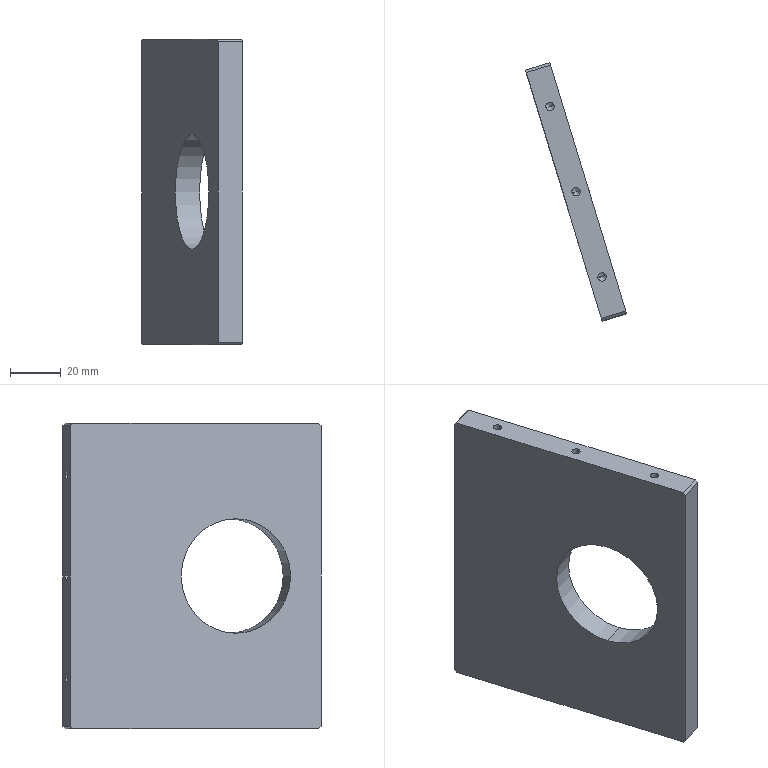Component | SolidWorks | V1ZHXTGrindingBasePlateReinforcementRibSB1-1 | 1 solid | 36 faces | box 39.62 x 101.43 x 120 mm | volume 107140 mm3 | cylinder 14 | cone 12 | plane 10 | commonest cylinder face diameters 3.3 x12 45 x2
build123d program:
from build123d import *

# Parameters (mm, degrees)
SKETCH1_W             = 120
SKETCH1_H             = 103
BOSS_EXTRUDE1_DEPTH   = 5
M4_TAPPED_HOLE1_D     = 3.3
M4_TAPPED_HOLE1_DEPTH = 10.1
M4_TAPPED_HOLE1_TIP   = 0.9914
M4_TAPPED_HOLE2_D     = 3.3
M4_TAPPED_HOLE2_DEPTH = 10.1
M4_TAPPED_HOLE2_TIP   = 0.9914
SKETCH7_R             = 22.5
CUT_EXTRUDE1_DEPTH    = 10
CHAMFER1_SIZE         = 1


with BuildPart() as part:
    # Sketch1 → Boss-Extrude1 (new, symmetric)
    with BuildSketch(Plane.XY):
        Rectangle(SKETCH1_W, SKETCH1_H)
    extrude(amount=BOSS_EXTRUDE1_DEPTH, both=True)

    # M4 Tapped Hole1
    with Locations(Plane.ZY.offset(60)):
        with Locations((0, 35), (0, 0), (0, -35)):
            Hole(M4_TAPPED_HOLE1_D / 2, depth=M4_TAPPED_HOLE1_DEPTH)
            with Locations((0, 0, -(M4_TAPPED_HOLE1_DEPTH + M4_TAPPED_HOLE1_TIP / 2))):  # 118° drill point
                Cone(0, M4_TAPPED_HOLE1_D / 2, M4_TAPPED_HOLE1_TIP, mode=Mode.SUBTRACT)

    # M4 Tapped Hole2
    with Locations(Plane(origin=(0, -51.5, 0), x_dir=(-1, 0, 0), z_dir=(0, -1, 0))):
        with Locations((40, 0), (0, 0), (-40, 0)):
            Hole(M4_TAPPED_HOLE2_D / 2, depth=M4_TAPPED_HOLE2_DEPTH)
            with Locations((0, 0, -(M4_TAPPED_HOLE2_DEPTH + M4_TAPPED_HOLE2_TIP / 2))):  # 118° drill point
                Cone(0, M4_TAPPED_HOLE2_D / 2, M4_TAPPED_HOLE2_TIP, mode=Mode.SUBTRACT)

    # Sketch7 → Cut-Extrude1 (cut)
    with BuildSketch(Plane.XY.offset(5)):
        with Locations((0, 16.5)):
            Circle(SKETCH7_R)
    extrude(amount=-CUT_EXTRUDE1_DEPTH, mode=Mode.SUBTRACT)

    # Chamfer1
    chamfer1_edges = [part.edges().sort_by_distance(p)[0] for p in [
        (60, -51.5, 0),
        (-60, -51.5, 0),
        (-60, 51.5, 0),
        (60, 51.5, 0),
    ]]
    chamfer(chamfer1_edges, length=CHAMFER1_SIZE)


solid = part.part

# Placed as in the assembly
solid = solid.moved(Location((244.147, -194.476, 375.239), (90, -73.032, -90)))
STEP:
#1=CARTESIAN_POINT('',(9.99,-8.22,15.659));
#2=VERTEX_POINT('',#1);
#3=CARTESIAN_POINT('',(9.99,-8.22,13.887));
#4=VERTEX_POINT('',#3);
#5=CARTESIAN_POINT('',(9.99,-8.22,14.773));
#6=DIRECTION('',(-0.9565,-0.2918,-0.));
#7=DIRECTION('',(0.,0.,-1.));
#8=AXIS2_PLACEMENT_3D('',#5,#6,#7);
#9=CIRCLE('',#8,0.8858);
#10=EDGE_CURVE('',#2,#4,#9,.T.);
#11=ORIENTED_EDGE('',*,*,#10,.F.);
#12=CARTESIAN_POINT('',(9.613,-8.335,15.659));
#13=VERTEX_POINT('',#12);
#14=CARTESIAN_POINT('',(9.99,-8.22,15.659));
#15=DIRECTION('',(-0.9565,-0.2918,-0.));
#16=VECTOR('',#15,39.37);
#17=LINE('',#14,#16);
#18=EDGE_CURVE('',#2,#13,#17,.T.);
#19=ORIENTED_EDGE('',*,*,#18,.T.);
#20=CARTESIAN_POINT('',(9.613,-8.335,13.887));
#21=VERTEX_POINT('',#20);
#22=CARTESIAN_POINT('',(9.613,-8.335,14.773));
#23=DIRECTION('',(-0.9565,-0.2918,-0.));
#24=DIRECTION('',(0.,0.,-1.));
#25=AXIS2_PLACEMENT_3D('',#22,#23,#24);
#26=CIRCLE('',#25,0.8858);
#27=EDGE_CURVE('',#13,#21,#26,.T.);
#28=ORIENTED_EDGE('',*,*,#27,.T.);
#29=CARTESIAN_POINT('',(9.99,-8.22,13.887));
#30=DIRECTION('',(-0.9565,-0.2918,-0.));
#31=VECTOR('',#30,39.37);
#32=LINE('',#29,#31);
#33=EDGE_CURVE('',#4,#21,#32,.T.);
#34=ORIENTED_EDGE('',*,*,#33,.F.);
#35=EDGE_LOOP('',(#11,#19,#28,#34));
#36=FACE_OUTER_BOUND('',#35,.T.);
#37=CARTESIAN_POINT('',(9.99,-8.22,14.773));
#38=DIRECTION('',(-0.9565,-0.2918,-0.));
#39=DIRECTION('',(0.,0.,-1.));
#40=AXIS2_PLACEMENT_3D('',#37,#38,#39);
#41=CYLINDRICAL_SURFACE('',#40,0.8858);
#42=ADVANCED_FACE('',(#36),#41,.F.);
#43=CARTESIAN_POINT('',(9.074,-6.117,16.348));
#44=VERTEX_POINT('',#43);
#45=CARTESIAN_POINT('',(9.199,-6.079,16.348));
#46=VERTEX_POINT('',#45);
#47=CARTESIAN_POINT('',(9.136,-6.098,16.348));
#48=DIRECTION('',(-0.2918,0.9565,0.));
#49=DIRECTION('',(0.9565,0.2918,0.));
#50=AXIS2_PLACEMENT_3D('',#47,#48,#49);
#51=CIRCLE('',#50,0.06496);
#52=EDGE_CURVE('',#44,#46,#51,.T.);
#53=ORIENTED_EDGE('',*,*,#52,.F.);
#54=CARTESIAN_POINT('',(8.958,-5.736,16.348));
#55=VERTEX_POINT('',#54);
#56=CARTESIAN_POINT('',(8.958,-5.736,16.348));
#57=DIRECTION('',(-0.2918,0.9565,0.));
#58=VECTOR('',#57,39.37);
#59=LINE('',#56,#58);
#60=EDGE_CURVE('',#44,#55,#59,.T.);
#61=ORIENTED_EDGE('',*,*,#60,.T.);
#62=CARTESIAN_POINT('',(9.083,-5.698,16.348));
#63=VERTEX_POINT('',#62);
#64=CARTESIAN_POINT('',(9.02,-5.717,16.348));
#65=DIRECTION('',(-0.2918,0.9565,0.));
#66=DIRECTION('',(0.9565,0.2918,0.));
#67=AXIS2_PLACEMENT_3D('',#64,#65,#66);
#68=CIRCLE('',#67,0.06496);
#69=EDGE_CURVE('',#55,#63,#68,.T.);
#70=ORIENTED_EDGE('',*,*,#69,.T.);
#71=CARTESIAN_POINT('',(9.083,-5.698,16.348));
#72=DIRECTION('',(-0.2918,0.9565,0.));
#73=VECTOR('',#72,39.37);
#74=LINE('',#71,#73);
#75=EDGE_CURVE('',#46,#63,#74,.T.);
#76=ORIENTED_EDGE('',*,*,#75,.F.);
#77=EDGE_LOOP('',(#53,#61,#70,#76));
#78=FACE_OUTER_BOUND('',#77,.T.);
#79=CARTESIAN_POINT('',(9.02,-5.717,16.348));
#80=DIRECTION('',(-0.2918,0.9565,0.));
#81=DIRECTION('',(0.9565,0.2918,0.));
#82=AXIS2_PLACEMENT_3D('',#79,#80,#81);
#83=CYLINDRICAL_SURFACE('',#82,0.06496);
#84=ADVANCED_FACE('',(#78),#83,.F.);
#85=CARTESIAN_POINT('',(9.148,-6.135,16.348));
#86=VERTEX_POINT('',#85);
#87=CARTESIAN_POINT('',(9.199,-6.079,16.348));
#88=DIRECTION('',(0.6696,0.7428,0.));
#89=VECTOR('',#88,39.37);
#90=LINE('',#87,#89);
#91=EDGE_CURVE('',#86,#46,#90,.T.);
#92=ORIENTED_EDGE('',*,*,#91,.F.);
#93=CARTESIAN_POINT('',(9.074,-6.117,16.348));
#94=DIRECTION('',(-0.9702,0.2425,0.));
#95=VECTOR('',#94,39.37);
#96=LINE('',#93,#95);
#97=EDGE_CURVE('',#86,#44,#96,.T.);
#98=ORIENTED_EDGE('',*,*,#97,.T.);
#99=ORIENTED_EDGE('',*,*,#52,.T.);
#100=EDGE_LOOP('',(#92,#98,#99));
#101=FACE_OUTER_BOUND('',#100,.T.);
#102=CARTESIAN_POINT('',(9.136,-6.098,16.348));
#103=DIRECTION('',(-0.2918,0.9565,0.));
#104=DIRECTION('',(0.9565,0.2918,0.));
#105=AXIS2_PLACEMENT_3D('',#102,#103,#104);
#106=CONICAL_SURFACE('',#105,0.06496,1.03);
#107=ADVANCED_FACE('',(#101),#106,.F.);
#108=CARTESIAN_POINT('',(9.074,-6.117,14.773));
#109=VERTEX_POINT('',#108);
#110=CARTESIAN_POINT('',(9.199,-6.079,14.773));
#111=VERTEX_POINT('',#110);
#112=CARTESIAN_POINT('',(9.136,-6.098,14.773));
#113=DIRECTION('',(-0.2918,0.9565,0.));
#114=DIRECTION('',(0.9565,0.2918,0.));
#115=AXIS2_PLACEMENT_3D('',#112,#113,#114);
#116=CIRCLE('',#115,0.06496);
#117=EDGE_CURVE('',#109,#111,#116,.T.);
#118=ORIENTED_EDGE('',*,*,#117,.F.);
#119=CARTESIAN_POINT('',(8.958,-5.736,14.773));
#120=VERTEX_POINT('',#119);
#121=CARTESIAN_POINT('',(8.958,-5.736,14.773));
#122=DIRECTION('',(-0.2918,0.9565,0.));
#123=VECTOR('',#122,39.37);
#124=LINE('',#121,#123);
#125=EDGE_CURVE('',#109,#120,#124,.T.);
#126=ORIENTED_EDGE('',*,*,#125,.T.);
#127=CARTESIAN_POINT('',(9.083,-5.698,14.773));
#128=VERTEX_POINT('',#127);
#129=CARTESIAN_POINT('',(9.02,-5.717,14.773));
#130=DIRECTION('',(-0.2918,0.9565,0.));
#131=DIRECTION('',(0.9565,0.2918,0.));
#132=AXIS2_PLACEMENT_3D('',#129,#130,#131);
#133=CIRCLE('',#132,0.06496);
#134=EDGE_CURVE('',#120,#128,#133,.T.);
#135=ORIENTED_EDGE('',*,*,#134,.T.);
#136=CARTESIAN_POINT('',(9.083,-5.698,14.773));
#137=DIRECTION('',(-0.2918,0.9565,0.));
#138=VECTOR('',#137,39.37);
#139=LINE('',#136,#138);
#140=EDGE_CURVE('',#111,#128,#139,.T.);
#141=ORIENTED_EDGE('',*,*,#140,.F.);
#142=EDGE_LOOP('',(#118,#126,#135,#141));
#143=FACE_OUTER_BOUND('',#142,.T.);
#144=CARTESIAN_POINT('',(9.02,-5.717,14.773));
#145=DIRECTION('',(-0.2918,0.9565,0.));
#146=DIRECTION('',(0.9565,0.2918,0.));
#147=AXIS2_PLACEMENT_3D('',#144,#145,#146);
#148=CYLINDRICAL_SURFACE('',#147,0.06496);
#149=ADVANCED_FACE('',(#143),#148,.F.);
#150=CARTESIAN_POINT('',(9.148,-6.135,14.773));
#151=VERTEX_POINT('',#150);
#152=CARTESIAN_POINT('',(9.199,-6.079,14.773));
#153=DIRECTION('',(0.6696,0.7428,0.));
#154=VECTOR('',#153,39.37);
#155=LINE('',#152,#154);
#156=EDGE_CURVE('',#151,#111,#155,.T.);
#157=ORIENTED_EDGE('',*,*,#156,.F.);
#158=CARTESIAN_POINT('',(9.074,-6.117,14.773));
#159=DIRECTION('',(-0.9702,0.2425,0.));
#160=VECTOR('',#159,39.37);
#161=LINE('',#158,#160);
#162=EDGE_CURVE('',#151,#109,#161,.T.);
#163=ORIENTED_EDGE('',*,*,#162,.T.);
#164=ORIENTED_EDGE('',*,*,#117,.T.);
#165=EDGE_LOOP('',(#157,#163,#164));
#166=FACE_OUTER_BOUND('',#165,.T.);
#167=CARTESIAN_POINT('',(9.136,-6.098,14.773));
#168=DIRECTION('',(-0.2918,0.9565,0.));
#169=DIRECTION('',(0.9565,0.2918,0.));
#170=AXIS2_PLACEMENT_3D('',#167,#168,#169);
#171=CONICAL_SURFACE('',#170,0.06496,1.03);
#172=ADVANCED_FACE('',(#166),#171,.F.);
#173=CARTESIAN_POINT('',(9.074,-6.117,13.198));
#174=VERTEX_POINT('',#173);
#175=CARTESIAN_POINT('',(9.199,-6.079,13.198));
#176=VERTEX_POINT('',#175);
#177=CARTESIAN_POINT('',(9.136,-6.098,13.198));
#178=DIRECTION('',(-0.2918,0.9565,0.));
#179=DIRECTION('',(0.9565,0.2918,0.));
#180=AXIS2_PLACEMENT_3D('',#177,#178,#179);
#181=CIRCLE('',#180,0.06496);
#182=EDGE_CURVE('',#174,#176,#181,.T.);
#183=ORIENTED_EDGE('',*,*,#182,.F.);
#184=CARTESIAN_POINT('',(8.958,-5.736,13.198));
#185=VERTEX_POINT('',#184);
#186=CARTESIAN_POINT('',(8.958,-5.736,13.198));
#187=DIRECTION('',(-0.2918,0.9565,0.));
#188=VECTOR('',#187,39.37);
#189=LINE('',#186,#188);
#190=EDGE_CURVE('',#174,#185,#189,.T.);
#191=ORIENTED_EDGE('',*,*,#190,.T.);
#192=CARTESIAN_POINT('',(9.083,-5.698,13.198));
#193=VERTEX_POINT('',#192);
#194=CARTESIAN_POINT('',(9.02,-5.717,13.198));
#195=DIRECTION('',(-0.2918,0.9565,0.));
#196=DIRECTION('',(0.9565,0.2918,0.));
#197=AXIS2_PLACEMENT_3D('',#194,#195,#196);
#198=CIRCLE('',#197,0.06496);
#199=EDGE_CURVE('',#185,#193,#198,.T.);
#200=ORIENTED_EDGE('',*,*,#199,.T.);
#201=CARTESIAN_POINT('',(9.083,-5.698,13.198));
#202=DIRECTION('',(-0.2918,0.9565,0.));
#203=VECTOR('',#202,39.37);
#204=LINE('',#201,#203);
#205=EDGE_CURVE('',#176,#193,#204,.T.);
#206=ORIENTED_EDGE('',*,*,#205,.F.);
#207=EDGE_LOOP('',(#183,#191,#200,#206));
#208=FACE_OUTER_BOUND('',#207,.T.);
#209=CARTESIAN_POINT('',(9.02,-5.717,13.198));
#210=DIRECTION('',(-0.2918,0.9565,0.));
#211=DIRECTION('',(0.9565,0.2918,0.));
#212=AXIS2_PLACEMENT_3D('',#209,#210,#211);
#213=CYLINDRICAL_SURFACE('',#212,0.06496);
#214=ADVANCED_FACE('',(#208),#213,.F.);
#215=CARTESIAN_POINT('',(9.148,-6.135,13.198));
#216=VERTEX_POINT('',#215);
#217=CARTESIAN_POINT('',(9.199,-6.079,13.198));
#218=DIRECTION('',(0.6696,0.7428,0.));
#219=VECTOR('',#218,39.37);
#220=LINE('',#217,#219);
#221=EDGE_CURVE('',#216,#176,#220,.T.);
#222=ORIENTED_EDGE('',*,*,#221,.F.);
#223=CARTESIAN_POINT('',(9.074,-6.117,13.198));
#224=DIRECTION('',(-0.9702,0.2425,0.));
#225=VECTOR('',#224,39.37);
#226=LINE('',#223,#225);
#227=EDGE_CURVE('',#216,#174,#226,.T.);
#228=ORIENTED_EDGE('',*,*,#227,.T.);
#229=ORIENTED_EDGE('',*,*,#182,.T.);
#230=EDGE_LOOP('',(#222,#228,#229));
#231=FACE_OUTER_BOUND('',#230,.T.);
#232=CARTESIAN_POINT('',(9.136,-6.098,13.198));
#233=DIRECTION('',(-0.2918,0.9565,0.));
#234=DIRECTION('',(0.9565,0.2918,0.));
#235=AXIS2_PLACEMENT_3D('',#232,#233,#234);
#236=CONICAL_SURFACE('',#235,0.06496,1.03);
#237=ADVANCED_FACE('',(#231),#236,.F.);
#238=CARTESIAN_POINT('',(10.076,-8.956,16.738));
#239=VERTEX_POINT('',#238);
#240=CARTESIAN_POINT('',(9.952,-8.993,16.738));
#241=VERTEX_POINT('',#240);
#242=CARTESIAN_POINT('',(10.014,-8.975,16.738));
#243=DIRECTION('',(-0.,-0.,1.));
#244=DIRECTION('',(-0.9565,-0.2918,-0.));
#245=AXIS2_PLACEMENT_3D('',#242,#243,#244);
#246=CIRCLE('',#245,0.06496);
#247=EDGE_CURVE('',#239,#241,#246,.T.);
#248=ORIENTED_EDGE('',*,*,#247,.F.);
#249=CARTESIAN_POINT('',(10.076,-8.956,17.135));
#250=VERTEX_POINT('',#249);
#251=CARTESIAN_POINT('',(10.076,-8.956,17.135));
#252=DIRECTION('',(-0.,-0.,1.));
#253=VECTOR('',#252,39.37);
#254=LINE('',#251,#253);
#255=EDGE_CURVE('',#239,#250,#254,.T.);
#256=ORIENTED_EDGE('',*,*,#255,.T.);
#257=CARTESIAN_POINT('',(9.952,-8.993,17.135));
#258=VERTEX_POINT('',#257);
#259=CARTESIAN_POINT('',(10.014,-8.975,17.135));
#260=DIRECTION('',(-0.,-0.,1.));
#261=DIRECTION('',(-0.9565,-0.2918,-0.));
#262=AXIS2_PLACEMENT_3D('',#259,#260,#261);
#263=CIRCLE('',#262,0.06496);
#264=EDGE_CURVE('',#250,#258,#263,.T.);
#265=ORIENTED_EDGE('',*,*,#264,.T.);
#266=CARTESIAN_POINT('',(9.952,-8.993,17.135));
#267=DIRECTION('',(-0.,-0.,1.));
#268=VECTOR('',#267,39.37);
#269=LINE('',#266,#268);
#270=EDGE_CURVE('',#241,#258,#269,.T.);
#271=ORIENTED_EDGE('',*,*,#270,.F.);
#272=EDGE_LOOP('',(#248,#256,#265,#271));
#273=FACE_OUTER_BOUND('',#272,.T.);
#274=CARTESIAN_POINT('',(10.014,-8.975,17.135));
#275=DIRECTION('',(-0.,-0.,1.));
#276=DIRECTION('',(-0.9565,-0.2918,-0.));
#277=AXIS2_PLACEMENT_3D('',#274,#275,#276);
#278=CYLINDRICAL_SURFACE('',#277,0.06496);
#279=ADVANCED_FACE('',(#273),#278,.F.);
#280=CARTESIAN_POINT('',(10.014,-8.975,16.699));
#281=VERTEX_POINT('',#280);
#282=CARTESIAN_POINT('',(9.952,-8.993,16.738));
#283=DIRECTION('',(-0.8199,-0.2501,0.515));
#284=VECTOR('',#283,39.37);
#285=LINE('',#282,#284);
#286=EDGE_CURVE('',#281,#241,#285,.T.);
#287=ORIENTED_EDGE('',*,*,#286,.F.);
#288=CARTESIAN_POINT('',(10.076,-8.956,16.738));
#289=DIRECTION('',(0.8199,0.2501,0.515));
#290=VECTOR('',#289,39.37);
#291=LINE('',#288,#290);
#292=EDGE_CURVE('',#281,#239,#291,.T.);
#293=ORIENTED_EDGE('',*,*,#292,.T.);
#294=ORIENTED_EDGE('',*,*,#247,.T.);
#295=EDGE_LOOP('',(#287,#293,#294));
#296=FACE_OUTER_BOUND('',#295,.T.);
#297=CARTESIAN_POINT('',(10.014,-8.975,16.738));
#298=DIRECTION('',(-0.,-0.,1.));
#299=DIRECTION('',(-0.9565,-0.2918,-0.));
#300=AXIS2_PLACEMENT_3D('',#297,#298,#299);
#301=CONICAL_SURFACE('',#300,0.06496,1.03);
#302=ADVANCED_FACE('',(#296),#301,.F.);
#303=CARTESIAN_POINT('',(9.674,-7.638,16.738));
#304=VERTEX_POINT('',#303);
#305=CARTESIAN_POINT('',(9.55,-7.675,16.738));
#306=VERTEX_POINT('',#305);
#307=CARTESIAN_POINT('',(9.612,-7.657,16.738));
#308=DIRECTION('',(-0.,-0.,1.));
#309=DIRECTION('',(-0.9565,-0.2918,-0.));
#310=AXIS2_PLACEMENT_3D('',#307,#308,#309);
#311=CIRCLE('',#310,0.06496);
#312=EDGE_CURVE('',#304,#306,#311,.T.);
#313=ORIENTED_EDGE('',*,*,#312,.F.);
#314=CARTESIAN_POINT('',(9.674,-7.638,17.135));
#315=VERTEX_POINT('',#314);
#316=CARTESIAN_POINT('',(9.674,-7.638,17.135));
#317=DIRECTION('',(-0.,-0.,1.));
#318=VECTOR('',#317,39.37);
#319=LINE('',#316,#318);
#320=EDGE_CURVE('',#304,#315,#319,.T.);
#321=ORIENTED_EDGE('',*,*,#320,.T.);
#322=CARTESIAN_POINT('',(9.55,-7.675,17.135));
#323=VERTEX_POINT('',#322);
#324=CARTESIAN_POINT('',(9.612,-7.657,17.135));
#325=DIRECTION('',(-0.,-0.,1.));
#326=DIRECTION('',(-0.9565,-0.2918,-0.));
#327=AXIS2_PLACEMENT_3D('',#324,#325,#326);
#328=CIRCLE('',#327,0.06496);
#329=EDGE_CURVE('',#315,#323,#328,.T.);
#330=ORIENTED_EDGE('',*,*,#329,.T.);
#331=CARTESIAN_POINT('',(9.55,-7.675,17.135));
#332=DIRECTION('',(-0.,-0.,1.));
#333=VECTOR('',#332,39.37);
#334=LINE('',#331,#333);
#335=EDGE_CURVE('',#306,#323,#334,.T.);
#336=ORIENTED_EDGE('',*,*,#335,.F.);
#337=EDGE_LOOP('',(#313,#321,#330,#336));
#338=FACE_OUTER_BOUND('',#337,.T.);
#339=CARTESIAN_POINT('',(9.612,-7.657,17.135));
#340=DIRECTION('',(-0.,-0.,1.));
#341=DIRECTION('',(-0.9565,-0.2918,-0.));
#342=AXIS2_PLACEMENT_3D('',#339,#340,#341);
#343=CYLINDRICAL_SURFACE('',#342,0.06496);
#344=ADVANCED_FACE('',(#338),#343,.F.);
#345=CARTESIAN_POINT('',(9.612,-7.657,16.699));
#346=VERTEX_POINT('',#345);
#347=CARTESIAN_POINT('',(9.55,-7.675,16.738));
#348=DIRECTION('',(-0.8199,-0.2501,0.515));
#349=VECTOR('',#348,39.37);
#350=LINE('',#347,#349);
#351=EDGE_CURVE('',#346,#306,#350,.T.);
#352=ORIENTED_EDGE('',*,*,#351,.F.);
#353=CARTESIAN_POINT('',(9.674,-7.638,16.738));
#354=DIRECTION('',(0.8199,0.2501,0.515));
#355=VECTOR('',#354,39.37);
#356=LINE('',#353,#355);
#357=EDGE_CURVE('',#346,#304,#356,.T.);
#358=ORIENTED_EDGE('',*,*,#357,.T.);
#359=ORIENTED_EDGE('',*,*,#312,.T.);
#360=EDGE_LOOP('',(#352,#358,#359));
#361=FACE_OUTER_BOUND('',#360,.T.);
#362=CARTESIAN_POINT('',(9.612,-7.657,16.738));
#363=DIRECTION('',(-0.,-0.,1.));
#364=DIRECTION('',(-0.9565,-0.2918,-0.));
#365=AXIS2_PLACEMENT_3D('',#362,#363,#364);
#366=CONICAL_SURFACE('',#365,0.06496,1.03);
#367=ADVANCED_FACE('',(#361),#366,.F.);
#368=CARTESIAN_POINT('',(9.272,-6.32,16.738));
#369=VERTEX_POINT('',#368);
#370=CARTESIAN_POINT('',(9.148,-6.358,16.738));
#371=VERTEX_POINT('',#370);
#372=CARTESIAN_POINT('',(9.21,-6.339,16.738));
#373=DIRECTION('',(-0.,-0.,1.));
#374=DIRECTION('',(-0.9565,-0.2918,-0.));
#375=AXIS2_PLACEMENT_3D('',#372,#373,#374);
#376=CIRCLE('',#375,0.06496);
#377=EDGE_CURVE('',#369,#371,#376,.T.);
#378=ORIENTED_EDGE('',*,*,#377,.F.);
#379=CARTESIAN_POINT('',(9.272,-6.32,17.135));
#380=VERTEX_POINT('',#379);
#381=CARTESIAN_POINT('',(9.272,-6.32,17.135));
#382=DIRECTION('',(-0.,-0.,1.));
#383=VECTOR('',#382,39.37);
#384=LINE('',#381,#383);
#385=EDGE_CURVE('',#369,#380,#384,.T.);
#386=ORIENTED_EDGE('',*,*,#385,.T.);
#387=CARTESIAN_POINT('',(9.148,-6.358,17.135));
#388=VERTEX_POINT('',#387);
#389=CARTESIAN_POINT('',(9.21,-6.339,17.135));
#390=DIRECTION('',(-0.,-0.,1.));
#391=DIRECTION('',(-0.9565,-0.2918,-0.));
#392=AXIS2_PLACEMENT_3D('',#389,#390,#391);
#393=CIRCLE('',#392,0.06496);
#394=EDGE_CURVE('',#380,#388,#393,.T.);
#395=ORIENTED_EDGE('',*,*,#394,.T.);
#396=CARTESIAN_POINT('',(9.148,-6.358,17.135));
#397=DIRECTION('',(-0.,-0.,1.));
#398=VECTOR('',#397,39.37);
#399=LINE('',#396,#398);
#400=EDGE_CURVE('',#371,#388,#399,.T.);
#401=ORIENTED_EDGE('',*,*,#400,.F.);
#402=EDGE_LOOP('',(#378,#386,#395,#401));
#403=FACE_OUTER_BOUND('',#402,.T.);
#404=CARTESIAN_POINT('',(9.21,-6.339,17.135));
#405=DIRECTION('',(-0.,-0.,1.));
#406=DIRECTION('',(-0.9565,-0.2918,-0.));
#407=AXIS2_PLACEMENT_3D('',#404,#405,#406);
#408=CYLINDRICAL_SURFACE('',#407,0.06496);
#409=ADVANCED_FACE('',(#403),#408,.F.);
#410=CARTESIAN_POINT('',(9.21,-6.339,16.699));
#411=VERTEX_POINT('',#410);
#412=CARTESIAN_POINT('',(9.148,-6.358,16.738));
#413=DIRECTION('',(-0.8199,-0.2501,0.515));
#414=VECTOR('',#413,39.37);
#415=LINE('',#412,#414);
#416=EDGE_CURVE('',#411,#371,#415,.T.);
#417=ORIENTED_EDGE('',*,*,#416,.F.);
#418=CARTESIAN_POINT('',(9.272,-6.32,16.738));
#419=DIRECTION('',(0.8199,0.2501,0.515));
#420=VECTOR('',#419,39.37);
#421=LINE('',#418,#420);
#422=EDGE_CURVE('',#411,#369,#421,.T.);
#423=ORIENTED_EDGE('',*,*,#422,.T.);
#424=ORIENTED_EDGE('',*,*,#377,.T.);
#425=EDGE_LOOP('',(#417,#423,#424));
#426=FACE_OUTER_BOUND('',#425,.T.);
#427=CARTESIAN_POINT('',(9.21,-6.339,16.738));
#428=DIRECTION('',(-0.,-0.,1.));
#429=DIRECTION('',(-0.9565,-0.2918,-0.));
#430=AXIS2_PLACEMENT_3D('',#427,#428,#429);
#431=CONICAL_SURFACE('',#430,0.06496,1.03);
#432=ADVANCED_FACE('',(#426),#431,.F.);
#433=CARTESIAN_POINT('',(9.22,-5.697,12.411));
#434=VERTEX_POINT('',#433);
#435=CARTESIAN_POINT('',(10.381,-9.501,12.411));
#436=VERTEX_POINT('',#435);
#437=CARTESIAN_POINT('',(9.209,-5.66,12.411));
#438=DIRECTION('',(0.2918,-0.9565,-0.));
#439=VECTOR('',#438,39.37);
#440=LINE('',#437,#439);
#441=EDGE_CURVE('',#434,#436,#440,.T.);
#442=ORIENTED_EDGE('',*,*,#441,.T.);
#443=CARTESIAN_POINT('',(10.004,-9.616,12.411));
#444=VERTEX_POINT('',#443);
#445=CARTESIAN_POINT('',(10.004,-9.616,12.411));
#446=DIRECTION('',(-0.9565,-0.2918,-0.));
#447=VECTOR('',#446,39.37);
#448=LINE('',#445,#447);
#449=EDGE_CURVE('',#436,#444,#448,.T.);
#450=ORIENTED_EDGE('',*,*,#449,.T.);
#451=CARTESIAN_POINT('',(8.844,-5.812,12.411));
#452=VERTEX_POINT('',#451);
#453=CARTESIAN_POINT('',(8.832,-5.775,12.411));
#454=DIRECTION('',(0.2918,-0.9565,-0.));
#455=VECTOR('',#454,39.37);
#456=LINE('',#453,#455);
#457=EDGE_CURVE('',#452,#444,#456,.T.);
#458=ORIENTED_EDGE('',*,*,#457,.F.);
#459=CARTESIAN_POINT('',(8.844,-5.812,12.411));
#460=DIRECTION('',(0.9565,0.2918,0.));
#461=VECTOR('',#460,39.37);
#462=LINE('',#459,#461);
#463=EDGE_CURVE('',#452,#434,#462,.T.);
#464=ORIENTED_EDGE('',*,*,#463,.T.);
#465=EDGE_LOOP('',(#442,#450,#458,#464));
#466=FACE_OUTER_BOUND('',#465,.T.);
#467=CARTESIAN_POINT('',(8.832,-5.775,12.411));
#468=DIRECTION('',(-0.,-0.,1.));
#469=DIRECTION('',(-0.9565,-0.2918,-0.));
#470=AXIS2_PLACEMENT_3D('',#467,#468,#469);
#471=PLANE('',#470);
#472=ADVANCED_FACE('',(#466),#471,.F.);
#473=CARTESIAN_POINT('',(10.392,-9.538,12.45));
#474=VERTEX_POINT('',#473);
#475=CARTESIAN_POINT('',(10.392,-9.538,17.096));
#476=VERTEX_POINT('',#475);
#477=CARTESIAN_POINT('',(10.392,-9.538,17.135));
#478=DIRECTION('',(-0.,-0.,1.));
#479=VECTOR('',#478,39.37);
#480=LINE('',#477,#479);
#481=EDGE_CURVE('',#474,#476,#480,.T.);
#482=ORIENTED_EDGE('',*,*,#481,.T.);
#483=CARTESIAN_POINT('',(10.016,-9.653,17.096));
#484=VERTEX_POINT('',#483);
#485=CARTESIAN_POINT('',(10.016,-9.653,17.096));
#486=DIRECTION('',(-0.9565,-0.2918,-0.));
#487=VECTOR('',#486,39.37);
#488=LINE('',#485,#487);
#489=EDGE_CURVE('',#476,#484,#488,.T.);
#490=ORIENTED_EDGE('',*,*,#489,.T.);
#491=CARTESIAN_POINT('',(10.016,-9.653,12.45));
#492=VERTEX_POINT('',#491);
#493=CARTESIAN_POINT('',(10.016,-9.653,17.135));
#494=DIRECTION('',(-0.,-0.,1.));
#495=VECTOR('',#494,39.37);
#496=LINE('',#493,#495);
#497=EDGE_CURVE('',#492,#484,#496,.T.);
#498=ORIENTED_EDGE('',*,*,#497,.F.);
#499=CARTESIAN_POINT('',(10.016,-9.653,12.45));
#500=DIRECTION('',(0.9565,0.2918,0.));
#501=VECTOR('',#500,39.37);
#502=LINE('',#499,#501);
#503=EDGE_CURVE('',#492,#474,#502,.T.);
#504=ORIENTED_EDGE('',*,*,#503,.T.);
#505=EDGE_LOOP('',(#482,#490,#498,#504));
#506=FACE_OUTER_BOUND('',#505,.T.);
#507=CARTESIAN_POINT('',(10.016,-9.653,17.135));
#508=DIRECTION('',(-0.2918,0.9565,0.));
#509=DIRECTION('',(0.9565,0.2918,0.));
#510=AXIS2_PLACEMENT_3D('',#507,#508,#509);
#511=PLANE('',#510);
#512=ADVANCED_FACE('',(#506),#511,.F.);
#513=CARTESIAN_POINT('',(10.014,-8.975,17.135));
#514=DIRECTION('',(-0.,-0.,1.));
#515=DIRECTION('',(-0.9565,-0.2918,-0.));
#516=AXIS2_PLACEMENT_3D('',#513,#514,#515);
#517=CIRCLE('',#516,0.06496);
#518=EDGE_CURVE('',#258,#250,#517,.T.);
#519=ORIENTED_EDGE('',*,*,#518,.F.);
#520=ORIENTED_EDGE('',*,*,#264,.F.);
#521=EDGE_LOOP('',(#519,#520));
#522=FACE_BOUND('',#521,.T.);
#523=CARTESIAN_POINT('',(9.612,-7.657,17.135));
#524=DIRECTION('',(-0.,-0.,1.));
#525=DIRECTION('',(-0.9565,-0.2918,-0.));
#526=AXIS2_PLACEMENT_3D('',#523,#524,#525);
#527=CIRCLE('',#526,0.06496);
#528=EDGE_CURVE('',#323,#315,#527,.T.);
#529=ORIENTED_EDGE('',*,*,#528,.F.);
#530=ORIENTED_EDGE('',*,*,#329,.F.);
#531=EDGE_LOOP('',(#529,#530));
#532=FACE_BOUND('',#531,.T.);
#533=CARTESIAN_POINT('',(9.21,-6.339,17.135));
#534=DIRECTION('',(-0.,-0.,1.));
#535=DIRECTION('',(-0.9565,-0.2918,-0.));
#536=AXIS2_PLACEMENT_3D('',#533,#534,#535);
#537=CIRCLE('',#536,0.06496);
#538=EDGE_CURVE('',#388,#380,#537,.T.);
#539=ORIENTED_EDGE('',*,*,#538,.F.);
#540=ORIENTED_EDGE('',*,*,#394,.F.);
#541=EDGE_LOOP('',(#539,#540));
#542=FACE_BOUND('',#541,.T.);
#543=CARTESIAN_POINT('',(10.004,-9.616,17.135));
#544=VERTEX_POINT('',#543);
#545=CARTESIAN_POINT('',(8.844,-5.812,17.135));
#546=VERTEX_POINT('',#545);
#547=CARTESIAN_POINT('',(8.832,-5.775,17.135));
#548=DIRECTION('',(-0.2918,0.9565,0.));
#549=VECTOR('',#548,39.37);
#550=LINE('',#547,#549);
#551=EDGE_CURVE('',#544,#546,#550,.T.);
#552=ORIENTED_EDGE('',*,*,#551,.F.);
#553=CARTESIAN_POINT('',(10.381,-9.501,17.135));
#554=VERTEX_POINT('',#553);
#555=CARTESIAN_POINT('',(10.004,-9.616,17.135));
#556=DIRECTION('',(0.9565,0.2918,0.));
#557=VECTOR('',#556,39.37);
#558=LINE('',#555,#557);
#559=EDGE_CURVE('',#544,#554,#558,.T.);
#560=ORIENTED_EDGE('',*,*,#559,.T.);
#561=CARTESIAN_POINT('',(9.22,-5.697,17.135));
#562=VERTEX_POINT('',#561);
#563=CARTESIAN_POINT('',(9.209,-5.66,17.135));
#564=DIRECTION('',(-0.2918,0.9565,0.));
#565=VECTOR('',#564,39.37);
#566=LINE('',#563,#565);
#567=EDGE_CURVE('',#554,#562,#566,.T.);
#568=ORIENTED_EDGE('',*,*,#567,.T.);
#569=CARTESIAN_POINT('',(8.844,-5.812,17.135));
#570=DIRECTION('',(-0.9565,-0.2918,-0.));
#571=VECTOR('',#570,39.37);
#572=LINE('',#569,#571);
#573=EDGE_CURVE('',#562,#546,#572,.T.);
#574=ORIENTED_EDGE('',*,*,#573,.T.);
#575=EDGE_LOOP('',(#552,#560,#568,#574));
#576=FACE_OUTER_BOUND('',#575,.T.);
#577=CARTESIAN_POINT('',(8.832,-5.775,17.135));
#578=DIRECTION('',(0.,0.,-1.));
#579=DIRECTION('',(0.9565,0.2918,0.));
#580=AXIS2_PLACEMENT_3D('',#577,#578,#579);
#581=PLANE('',#580);
#582=ADVANCED_FACE('',(#522,#532,#542,#576),#581,.F.);
#583=CARTESIAN_POINT('',(9.02,-5.717,16.348));
#584=DIRECTION('',(-0.2918,0.9565,0.));
#585=DIRECTION('',(0.9565,0.2918,0.));
#586=AXIS2_PLACEMENT_3D('',#583,#584,#585);
#587=CIRCLE('',#586,0.06496);
#588=EDGE_CURVE('',#63,#55,#587,.T.);
#589=ORIENTED_EDGE('',*,*,#588,.F.);
#590=ORIENTED_EDGE('',*,*,#69,.F.);
#591=EDGE_LOOP('',(#589,#590));
#592=FACE_BOUND('',#591,.T.);
#593=CARTESIAN_POINT('',(9.02,-5.717,14.773));
#594=DIRECTION('',(-0.2918,0.9565,0.));
#595=DIRECTION('',(0.9565,0.2918,0.));
#596=AXIS2_PLACEMENT_3D('',#593,#594,#595);
#597=CIRCLE('',#596,0.06496);
#598=EDGE_CURVE('',#128,#120,#597,.T.);
#599=ORIENTED_EDGE('',*,*,#598,.F.);
#600=ORIENTED_EDGE('',*,*,#134,.F.);
#601=EDGE_LOOP('',(#599,#600));
#602=FACE_BOUND('',#601,.T.);
#603=CARTESIAN_POINT('',(9.02,-5.717,13.198));
#604=DIRECTION('',(-0.2918,0.9565,0.));
#605=DIRECTION('',(0.9565,0.2918,0.));
#606=AXIS2_PLACEMENT_3D('',#603,#604,#605);
#607=CIRCLE('',#606,0.06496);
#608=EDGE_CURVE('',#193,#185,#607,.T.);
#609=ORIENTED_EDGE('',*,*,#608,.F.);
#610=ORIENTED_EDGE('',*,*,#199,.F.);
#611=EDGE_LOOP('',(#609,#610));
#612=FACE_BOUND('',#611,.T.);
#613=CARTESIAN_POINT('',(9.209,-5.66,17.096));
#614=VERTEX_POINT('',#613);
#615=CARTESIAN_POINT('',(9.209,-5.66,12.45));
#616=VERTEX_POINT('',#615);
#617=CARTESIAN_POINT('',(9.209,-5.66,17.135));
#618=DIRECTION('',(0.,0.,-1.));
#619=VECTOR('',#618,39.37);
#620=LINE('',#617,#619);
#621=EDGE_CURVE('',#614,#616,#620,.T.);
#622=ORIENTED_EDGE('',*,*,#621,.T.);
#623=CARTESIAN_POINT('',(8.832,-5.775,12.45));
#624=VERTEX_POINT('',#623);
#625=CARTESIAN_POINT('',(8.832,-5.775,12.45));
#626=DIRECTION('',(-0.9565,-0.2918,-0.));
#627=VECTOR('',#626,39.37);
#628=LINE('',#625,#627);
#629=EDGE_CURVE('',#616,#624,#628,.T.);
#630=ORIENTED_EDGE('',*,*,#629,.T.);
#631=CARTESIAN_POINT('',(8.832,-5.775,17.096));
#632=VERTEX_POINT('',#631);
#633=CARTESIAN_POINT('',(8.832,-5.775,17.135));
#634=DIRECTION('',(0.,0.,-1.));
#635=VECTOR('',#634,39.37);
#636=LINE('',#633,#635);
#637=EDGE_CURVE('',#632,#624,#636,.T.);
#638=ORIENTED_EDGE('',*,*,#637,.F.);
#639=CARTESIAN_POINT('',(8.832,-5.775,17.096));
#640=DIRECTION('',(0.9565,0.2918,0.));
#641=VECTOR('',#640,39.37);
#642=LINE('',#639,#641);
#643=EDGE_CURVE('',#632,#614,#642,.T.);
#644=ORIENTED_EDGE('',*,*,#643,.T.);
#645=EDGE_LOOP('',(#622,#630,#638,#644));
#646=FACE_OUTER_BOUND('',#645,.T.);
#647=CARTESIAN_POINT('',(8.832,-5.775,17.135));
#648=DIRECTION('',(0.2918,-0.9565,-0.));
#649=DIRECTION('',(-0.9565,-0.2918,-0.));
#650=AXIS2_PLACEMENT_3D('',#647,#648,#649);
#651=PLANE('',#650);
#652=ADVANCED_FACE('',(#592,#602,#612,#646),#651,.F.);
#653=CARTESIAN_POINT('',(9.613,-8.335,14.773));
#654=DIRECTION('',(-0.9565,-0.2918,-0.));
#655=DIRECTION('',(0.,0.,-1.));
#656=AXIS2_PLACEMENT_3D('',#653,#654,#655);
#657=CIRCLE('',#656,0.8858);
#658=EDGE_CURVE('',#21,#13,#657,.T.);
#659=ORIENTED_EDGE('',*,*,#658,.F.);
#660=ORIENTED_EDGE('',*,*,#27,.F.);
#661=EDGE_LOOP('',(#659,#660));
#662=FACE_BOUND('',#661,.T.);
#663=ORIENTED_EDGE('',*,*,#497,.T.);
#664=CARTESIAN_POINT('',(10.004,-9.616,17.135));
#665=DIRECTION('',(-0.2064,0.6763,0.7071));
#666=VECTOR('',#665,39.37);
#667=LINE('',#664,#666);
#668=EDGE_CURVE('',#484,#544,#667,.T.);
#669=ORIENTED_EDGE('',*,*,#668,.T.);
#670=ORIENTED_EDGE('',*,*,#551,.T.);
#671=CARTESIAN_POINT('',(8.832,-5.775,17.096));
#672=DIRECTION('',(-0.2064,0.6763,-0.7071));
#673=VECTOR('',#672,39.37);
#674=LINE('',#671,#673);
#675=EDGE_CURVE('',#546,#632,#674,.T.);
#676=ORIENTED_EDGE('',*,*,#675,.T.);
#677=ORIENTED_EDGE('',*,*,#637,.T.);
#678=CARTESIAN_POINT('',(8.844,-5.812,12.411));
#679=DIRECTION('',(0.2064,-0.6763,-0.7071));
#680=VECTOR('',#679,39.37);
#681=LINE('',#678,#680);
#682=EDGE_CURVE('',#624,#452,#681,.T.);
#683=ORIENTED_EDGE('',*,*,#682,.T.);
#684=ORIENTED_EDGE('',*,*,#457,.T.);
#685=CARTESIAN_POINT('',(10.016,-9.653,12.45));
#686=DIRECTION('',(0.2064,-0.6763,0.7071));
#687=VECTOR('',#686,39.37);
#688=LINE('',#685,#687);
#689=EDGE_CURVE('',#444,#492,#688,.T.);
#690=ORIENTED_EDGE('',*,*,#689,.T.);
#691=EDGE_LOOP('',(#663,#669,#670,#676,#677,#683,#684,#690));
#692=FACE_OUTER_BOUND('',#691,.T.);
#693=CARTESIAN_POINT('',(9.424,-7.714,14.773));
#694=DIRECTION('',(0.9565,0.2918,0.));
#695=DIRECTION('',(-0.,-0.,1.));
#696=AXIS2_PLACEMENT_3D('',#693,#694,#695);
#697=PLANE('',#696);
#698=ADVANCED_FACE('',(#662,#692),#697,.F.);
#699=CARTESIAN_POINT('',(9.99,-8.22,14.773));
#700=DIRECTION('',(-0.9565,-0.2918,-0.));
#701=DIRECTION('',(0.,0.,-1.));
#702=AXIS2_PLACEMENT_3D('',#699,#700,#701);
#703=CIRCLE('',#702,0.8858);
#704=EDGE_CURVE('',#4,#2,#703,.T.);
#705=ORIENTED_EDGE('',*,*,#704,.T.);
#706=ORIENTED_EDGE('',*,*,#10,.T.);
#707=EDGE_LOOP('',(#705,#706));
#708=FACE_BOUND('',#707,.T.);
#709=ORIENTED_EDGE('',*,*,#567,.F.);
#710=CARTESIAN_POINT('',(10.435,-9.68,16.948));
#711=DIRECTION('',(0.2064,-0.6763,-0.7071));
#712=VECTOR('',#711,39.37);
#713=LINE('',#710,#712);
#714=EDGE_CURVE('',#554,#476,#713,.T.);
#715=ORIENTED_EDGE('',*,*,#714,.T.);
#716=ORIENTED_EDGE('',*,*,#481,.F.);
#717=CARTESIAN_POINT('',(10.435,-9.68,12.598));
#718=DIRECTION('',(-0.2064,0.6763,-0.7071));
#719=VECTOR('',#718,39.37);
#720=LINE('',#717,#719);
#721=EDGE_CURVE('',#474,#436,#720,.T.);
#722=ORIENTED_EDGE('',*,*,#721,.T.);
#723=ORIENTED_EDGE('',*,*,#441,.F.);
#724=CARTESIAN_POINT('',(9.166,-5.519,12.598));
#725=DIRECTION('',(-0.2064,0.6763,0.7071));
#726=VECTOR('',#725,39.37);
#727=LINE('',#724,#726);
#728=EDGE_CURVE('',#434,#616,#727,.T.);
#729=ORIENTED_EDGE('',*,*,#728,.T.);
#730=ORIENTED_EDGE('',*,*,#621,.F.);
#731=CARTESIAN_POINT('',(9.166,-5.519,16.948));
#732=DIRECTION('',(0.2064,-0.6763,0.7071));
#733=VECTOR('',#732,39.37);
#734=LINE('',#731,#733);
#735=EDGE_CURVE('',#614,#562,#734,.T.);
#736=ORIENTED_EDGE('',*,*,#735,.T.);
#737=EDGE_LOOP('',(#709,#715,#716,#722,#723,#729,#730,#736));
#738=FACE_OUTER_BOUND('',#737,.T.);
#739=CARTESIAN_POINT('',(9.8,-7.599,14.773));
#740=DIRECTION('',(0.9565,0.2918,0.));
#741=DIRECTION('',(-0.,-0.,1.));
#742=AXIS2_PLACEMENT_3D('',#739,#740,#741);
#743=PLANE('',#742);
#744=ADVANCED_FACE('',(#708,#738),#743,.T.);
#745=ORIENTED_EDGE('',*,*,#422,.F.);
#746=ORIENTED_EDGE('',*,*,#416,.T.);
#747=CARTESIAN_POINT('',(9.21,-6.339,16.738));
#748=DIRECTION('',(-0.,-0.,1.));
#749=DIRECTION('',(-0.9565,-0.2918,-0.));
#750=AXIS2_PLACEMENT_3D('',#747,#748,#749);
#751=CIRCLE('',#750,0.06496);
#752=EDGE_CURVE('',#371,#369,#751,.T.);
#753=ORIENTED_EDGE('',*,*,#752,.T.);
#754=EDGE_LOOP('',(#745,#746,#753));
#755=FACE_OUTER_BOUND('',#754,.T.);
#756=CARTESIAN_POINT('',(9.21,-6.339,16.738));
#757=DIRECTION('',(-0.,-0.,1.));
#758=DIRECTION('',(-0.9565,-0.2918,-0.));
#759=AXIS2_PLACEMENT_3D('',#756,#757,#758);
#760=CONICAL_SURFACE('',#759,0.06496,1.03);
#761=ADVANCED_FACE('',(#755),#760,.F.);
#762=ORIENTED_EDGE('',*,*,#385,.F.);
#763=ORIENTED_EDGE('',*,*,#752,.F.);
#764=ORIENTED_EDGE('',*,*,#400,.T.);
#765=ORIENTED_EDGE('',*,*,#538,.T.);
#766=EDGE_LOOP('',(#762,#763,#764,#765));
#767=FACE_OUTER_BOUND('',#766,.T.);
#768=CARTESIAN_POINT('',(9.21,-6.339,17.135));
#769=DIRECTION('',(-0.,-0.,1.));
#770=DIRECTION('',(-0.9565,-0.2918,-0.));
#771=AXIS2_PLACEMENT_3D('',#768,#769,#770);
#772=CYLINDRICAL_SURFACE('',#771,0.06496);
#773=ADVANCED_FACE('',(#767),#772,.F.);
#774=ORIENTED_EDGE('',*,*,#357,.F.);
#775=ORIENTED_EDGE('',*,*,#351,.T.);
#776=CARTESIAN_POINT('',(9.612,-7.657,16.738));
#777=DIRECTION('',(-0.,-0.,1.));
#778=DIRECTION('',(-0.9565,-0.2918,-0.));
#779=AXIS2_PLACEMENT_3D('',#776,#777,#778);
#780=CIRCLE('',#779,0.06496);
#781=EDGE_CURVE('',#306,#304,#780,.T.);
#782=ORIENTED_EDGE('',*,*,#781,.T.);
#783=EDGE_LOOP('',(#774,#775,#782));
#784=FACE_OUTER_BOUND('',#783,.T.);
#785=CARTESIAN_POINT('',(9.612,-7.657,16.738));
#786=DIRECTION('',(-0.,-0.,1.));
#787=DIRECTION('',(-0.9565,-0.2918,-0.));
#788=AXIS2_PLACEMENT_3D('',#785,#786,#787);
#789=CONICAL_SURFACE('',#788,0.06496,1.03);
#790=ADVANCED_FACE('',(#784),#789,.F.);
#791=ORIENTED_EDGE('',*,*,#320,.F.);
#792=ORIENTED_EDGE('',*,*,#781,.F.);
#793=ORIENTED_EDGE('',*,*,#335,.T.);
#794=ORIENTED_EDGE('',*,*,#528,.T.);
#795=EDGE_LOOP('',(#791,#792,#793,#794));
#796=FACE_OUTER_BOUND('',#795,.T.);
#797=CARTESIAN_POINT('',(9.612,-7.657,17.135));
#798=DIRECTION('',(-0.,-0.,1.));
#799=DIRECTION('',(-0.9565,-0.2918,-0.));
#800=AXIS2_PLACEMENT_3D('',#797,#798,#799);
#801=CYLINDRICAL_SURFACE('',#800,0.06496);
#802=ADVANCED_FACE('',(#796),#801,.F.);
#803=ORIENTED_EDGE('',*,*,#292,.F.);
#804=ORIENTED_EDGE('',*,*,#286,.T.);
#805=CARTESIAN_POINT('',(10.014,-8.975,16.738));
#806=DIRECTION('',(-0.,-0.,1.));
#807=DIRECTION('',(-0.9565,-0.2918,-0.));
#808=AXIS2_PLACEMENT_3D('',#805,#806,#807);
#809=CIRCLE('',#808,0.06496);
#810=EDGE_CURVE('',#241,#239,#809,.T.);
#811=ORIENTED_EDGE('',*,*,#810,.T.);
#812=EDGE_LOOP('',(#803,#804,#811));
#813=FACE_OUTER_BOUND('',#812,.T.);
#814=CARTESIAN_POINT('',(10.014,-8.975,16.738));
#815=DIRECTION('',(-0.,-0.,1.));
#816=DIRECTION('',(-0.9565,-0.2918,-0.));
#817=AXIS2_PLACEMENT_3D('',#814,#815,#816);
#818=CONICAL_SURFACE('',#817,0.06496,1.03);
#819=ADVANCED_FACE('',(#813),#818,.F.);
#820=ORIENTED_EDGE('',*,*,#255,.F.);
#821=ORIENTED_EDGE('',*,*,#810,.F.);
#822=ORIENTED_EDGE('',*,*,#270,.T.);
#823=ORIENTED_EDGE('',*,*,#518,.T.);
#824=EDGE_LOOP('',(#820,#821,#822,#823));
#825=FACE_OUTER_BOUND('',#824,.T.);
#826=CARTESIAN_POINT('',(10.014,-8.975,17.135));
#827=DIRECTION('',(-0.,-0.,1.));
#828=DIRECTION('',(-0.9565,-0.2918,-0.));
#829=AXIS2_PLACEMENT_3D('',#826,#827,#828);
#830=CYLINDRICAL_SURFACE('',#829,0.06496);
#831=ADVANCED_FACE('',(#825),#830,.F.);
#832=ORIENTED_EDGE('',*,*,#227,.F.);
#833=ORIENTED_EDGE('',*,*,#221,.T.);
#834=CARTESIAN_POINT('',(9.136,-6.098,13.198));
#835=DIRECTION('',(-0.2918,0.9565,0.));
#836=DIRECTION('',(0.9565,0.2918,0.));
#837=AXIS2_PLACEMENT_3D('',#834,#835,#836);
#838=CIRCLE('',#837,0.06496);
#839=EDGE_CURVE('',#176,#174,#838,.T.);
#840=ORIENTED_EDGE('',*,*,#839,.T.);
#841=EDGE_LOOP('',(#832,#833,#840));
#842=FACE_OUTER_BOUND('',#841,.T.);
#843=CARTESIAN_POINT('',(9.136,-6.098,13.198));
#844=DIRECTION('',(-0.2918,0.9565,0.));
#845=DIRECTION('',(0.9565,0.2918,0.));
#846=AXIS2_PLACEMENT_3D('',#843,#844,#845);
#847=CONICAL_SURFACE('',#846,0.06496,1.03);
#848=ADVANCED_FACE('',(#842),#847,.F.);
#849=ORIENTED_EDGE('',*,*,#190,.F.);
#850=ORIENTED_EDGE('',*,*,#839,.F.);
#851=ORIENTED_EDGE('',*,*,#205,.T.);
#852=ORIENTED_EDGE('',*,*,#608,.T.);
#853=EDGE_LOOP('',(#849,#850,#851,#852));
#854=FACE_OUTER_BOUND('',#853,.T.);
#855=CARTESIAN_POINT('',(9.02,-5.717,13.198));
#856=DIRECTION('',(-0.2918,0.9565,0.));
#857=DIRECTION('',(0.9565,0.2918,0.));
#858=AXIS2_PLACEMENT_3D('',#855,#856,#857);
#859=CYLINDRICAL_SURFACE('',#858,0.06496);
#860=ADVANCED_FACE('',(#854),#859,.F.);
#861=ORIENTED_EDGE('',*,*,#162,.F.);
#862=ORIENTED_EDGE('',*,*,#156,.T.);
#863=CARTESIAN_POINT('',(9.136,-6.098,14.773));
#864=DIRECTION('',(-0.2918,0.9565,0.));
#865=DIRECTION('',(0.9565,0.2918,0.));
#866=AXIS2_PLACEMENT_3D('',#863,#864,#865);
#867=CIRCLE('',#866,0.06496);
#868=EDGE_CURVE('',#111,#109,#867,.T.);
#869=ORIENTED_EDGE('',*,*,#868,.T.);
#870=EDGE_LOOP('',(#861,#862,#869));
#871=FACE_OUTER_BOUND('',#870,.T.);
#872=CARTESIAN_POINT('',(9.136,-6.098,14.773));
#873=DIRECTION('',(-0.2918,0.9565,0.));
#874=DIRECTION('',(0.9565,0.2918,0.));
#875=AXIS2_PLACEMENT_3D('',#872,#873,#874);
#876=CONICAL_SURFACE('',#875,0.06496,1.03);
#877=ADVANCED_FACE('',(#871),#876,.F.);
#878=ORIENTED_EDGE('',*,*,#125,.F.);
#879=ORIENTED_EDGE('',*,*,#868,.F.);
#880=ORIENTED_EDGE('',*,*,#140,.T.);
#881=ORIENTED_EDGE('',*,*,#598,.T.);
#882=EDGE_LOOP('',(#878,#879,#880,#881));
#883=FACE_OUTER_BOUND('',#882,.T.);
#884=CARTESIAN_POINT('',(9.02,-5.717,14.773));
#885=DIRECTION('',(-0.2918,0.9565,0.));
#886=DIRECTION('',(0.9565,0.2918,0.));
#887=AXIS2_PLACEMENT_3D('',#884,#885,#886);
#888=CYLINDRICAL_SURFACE('',#887,0.06496);
#889=ADVANCED_FACE('',(#883),#888,.F.);
#890=ORIENTED_EDGE('',*,*,#97,.F.);
#891=ORIENTED_EDGE('',*,*,#91,.T.);
#892=CARTESIAN_POINT('',(9.136,-6.098,16.348));
#893=DIRECTION('',(-0.2918,0.9565,0.));
#894=DIRECTION('',(0.9565,0.2918,0.));
#895=AXIS2_PLACEMENT_3D('',#892,#893,#894);
#896=CIRCLE('',#895,0.06496);
#897=EDGE_CURVE('',#46,#44,#896,.T.);
#898=ORIENTED_EDGE('',*,*,#897,.T.);
#899=EDGE_LOOP('',(#890,#891,#898));
#900=FACE_OUTER_BOUND('',#899,.T.);
#901=CARTESIAN_POINT('',(9.136,-6.098,16.348));
#902=DIRECTION('',(-0.2918,0.9565,0.));
#903=DIRECTION('',(0.9565,0.2918,0.));
#904=AXIS2_PLACEMENT_3D('',#901,#902,#903);
#905=CONICAL_SURFACE('',#904,0.06496,1.03);
#906=ADVANCED_FACE('',(#900),#905,.F.);
#907=ORIENTED_EDGE('',*,*,#60,.F.);
#908=ORIENTED_EDGE('',*,*,#897,.F.);
#909=ORIENTED_EDGE('',*,*,#75,.T.);
#910=ORIENTED_EDGE('',*,*,#588,.T.);
#911=EDGE_LOOP('',(#907,#908,#909,#910));
#912=FACE_OUTER_BOUND('',#911,.T.);
#913=CARTESIAN_POINT('',(9.02,-5.717,16.348));
#914=DIRECTION('',(-0.2918,0.9565,0.));
#915=DIRECTION('',(0.9565,0.2918,0.));
#916=AXIS2_PLACEMENT_3D('',#913,#914,#915);
#917=CYLINDRICAL_SURFACE('',#916,0.06496);
#918=ADVANCED_FACE('',(#912),#917,.F.);
#919=ORIENTED_EDGE('',*,*,#18,.F.);
#920=ORIENTED_EDGE('',*,*,#704,.F.);
#921=ORIENTED_EDGE('',*,*,#33,.T.);
#922=ORIENTED_EDGE('',*,*,#658,.T.);
#923=EDGE_LOOP('',(#919,#920,#921,#922));
#924=FACE_OUTER_BOUND('',#923,.T.);
#925=CARTESIAN_POINT('',(9.99,-8.22,14.773));
#926=DIRECTION('',(-0.9565,-0.2918,-0.));
#927=DIRECTION('',(0.,0.,-1.));
#928=AXIS2_PLACEMENT_3D('',#925,#926,#927);
#929=CYLINDRICAL_SURFACE('',#928,0.8858);
#930=ADVANCED_FACE('',(#924),#929,.F.);
#931=ORIENTED_EDGE('',*,*,#668,.F.);
#932=ORIENTED_EDGE('',*,*,#489,.F.);
#933=ORIENTED_EDGE('',*,*,#714,.F.);
#934=ORIENTED_EDGE('',*,*,#559,.F.);
#935=EDGE_LOOP('',(#931,#932,#933,#934));
#936=FACE_OUTER_BOUND('',#935,.T.);
#937=CARTESIAN_POINT('',(10.004,-9.616,17.135));
#938=DIRECTION('',(-0.2064,0.6763,-0.7071));
#939=DIRECTION('',(0.9565,0.2918,0.));
#940=AXIS2_PLACEMENT_3D('',#937,#938,#939);
#941=PLANE('',#940);
#942=ADVANCED_FACE('',(#936),#941,.F.);
#943=ORIENTED_EDGE('',*,*,#689,.F.);
#944=ORIENTED_EDGE('',*,*,#449,.F.);
#945=ORIENTED_EDGE('',*,*,#721,.F.);
#946=ORIENTED_EDGE('',*,*,#503,.F.);
#947=EDGE_LOOP('',(#943,#944,#945,#946));
#948=FACE_OUTER_BOUND('',#947,.T.);
#949=CARTESIAN_POINT('',(10.016,-9.653,12.45));
#950=DIRECTION('',(-0.2064,0.6763,0.7071));
#951=DIRECTION('',(0.9565,0.2918,0.));
#952=AXIS2_PLACEMENT_3D('',#949,#950,#951);
#953=PLANE('',#952);
#954=ADVANCED_FACE('',(#948),#953,.F.);
#955=ORIENTED_EDGE('',*,*,#682,.F.);
#956=ORIENTED_EDGE('',*,*,#629,.F.);
#957=ORIENTED_EDGE('',*,*,#728,.F.);
#958=ORIENTED_EDGE('',*,*,#463,.F.);
#959=EDGE_LOOP('',(#955,#956,#957,#958));
#960=FACE_OUTER_BOUND('',#959,.T.);
#961=CARTESIAN_POINT('',(8.844,-5.812,12.411));
#962=DIRECTION('',(0.2064,-0.6763,0.7071));
#963=DIRECTION('',(0.9565,0.2918,0.));
#964=AXIS2_PLACEMENT_3D('',#961,#962,#963);
#965=PLANE('',#964);
#966=ADVANCED_FACE('',(#960),#965,.F.);
#967=ORIENTED_EDGE('',*,*,#675,.F.);
#968=ORIENTED_EDGE('',*,*,#573,.F.);
#969=ORIENTED_EDGE('',*,*,#735,.F.);
#970=ORIENTED_EDGE('',*,*,#643,.F.);
#971=EDGE_LOOP('',(#967,#968,#969,#970));
#972=FACE_OUTER_BOUND('',#971,.T.);
#973=CARTESIAN_POINT('',(8.832,-5.775,17.096));
#974=DIRECTION('',(0.2064,-0.6763,-0.7071));
#975=DIRECTION('',(0.9565,0.2918,0.));
#976=AXIS2_PLACEMENT_3D('',#973,#974,#975);
#977=PLANE('',#976);
#978=ADVANCED_FACE('',(#972),#977,.F.);
#979=CLOSED_SHELL('',(#42,#84,#107,#149,#172,#214,#237,#279,#302,#344,#367,#409,#432,#472,#512,#582,#652,#698,#744,#761,#773,#790,#802,#819,#831,#848,#860,#877,#889,#906,#918,#930,#942,#954,#966,#978));
#980=MANIFOLD_SOLID_BREP('',#979);
#981=CARTESIAN_POINT('',(0.,0.,0.));
#982=DIRECTION('',(0.,0.,1.));
#983=DIRECTION('',(1.,0.,0.));
#984=AXIS2_PLACEMENT_3D('',#981,#982,#983);
#985=(LENGTH_UNIT()NAMED_UNIT(*)SI_UNIT($,.METRE.));
#986=LENGTH_MEASURE_WITH_UNIT(LENGTH_MEASURE(0.0254),#985);
#987=DIMENSIONAL_EXPONENTS(1.,0.,0.,0.,0.,0.,0.);
#988=(CONVERSION_BASED_UNIT('',#986)LENGTH_UNIT()NAMED_UNIT(#987));
#989=UNCERTAINTY_MEASURE_WITH_UNIT(LENGTH_MEASURE(0.00001),#988,'','');
#990=(NAMED_UNIT(*)PLANE_ANGLE_UNIT()SI_UNIT($,.RADIAN.));
#991=(NAMED_UNIT(*)SI_UNIT($,.STERADIAN.)SOLID_ANGLE_UNIT());
#992=(GEOMETRIC_REPRESENTATION_CONTEXT(3)GLOBAL_UNCERTAINTY_ASSIGNED_CONTEXT((#989))GLOBAL_UNIT_ASSIGNED_CONTEXT((#988,#990,#991))REPRESENTATION_CONTEXT('',''));
#993=ADVANCED_BREP_SHAPE_REPRESENTATION('',(#980,#984),#992);
#994=COLOUR_RGB('',0.7922,0.8196,0.9333);
#995=FILL_AREA_STYLE_COLOUR('',#994);
#996=FILL_AREA_STYLE('',(#995));
#997=SURFACE_STYLE_FILL_AREA(#996);
#998=SURFACE_SIDE_STYLE('',(#997));
#999=SURFACE_STYLE_USAGE(.BOTH.,#998);
#1000=PRESENTATION_STYLE_ASSIGNMENT((#999));
#1001=STYLED_ITEM('',(#1000),#980);
#1002=PRESENTATION_LAYER_ASSIGNMENT('','',(#1001));
#1003=(LENGTH_UNIT()NAMED_UNIT(*)SI_UNIT($,.METRE.));
#1004=LENGTH_MEASURE_WITH_UNIT(LENGTH_MEASURE(0.0254),#1003);
#1005=DIMENSIONAL_EXPONENTS(1.,0.,0.,0.,0.,0.,0.);
#1006=(CONVERSION_BASED_UNIT('',#1004)LENGTH_UNIT()NAMED_UNIT(#1005));
#1007=UNCERTAINTY_MEASURE_WITH_UNIT(LENGTH_MEASURE(0.00001),#1006,'','');
#1008=(NAMED_UNIT(*)PLANE_ANGLE_UNIT()SI_UNIT($,.RADIAN.));
#1009=(NAMED_UNIT(*)SI_UNIT($,.STERADIAN.)SOLID_ANGLE_UNIT());
#1010=(GEOMETRIC_REPRESENTATION_CONTEXT(3)GLOBAL_UNCERTAINTY_ASSIGNED_CONTEXT((#1007))GLOBAL_UNIT_ASSIGNED_CONTEXT((#1006,#1008,#1009))REPRESENTATION_CONTEXT('',''));
#1011=MECHANICAL_DESIGN_GEOMETRIC_PRESENTATION_REPRESENTATION('',(#1001),#1010);